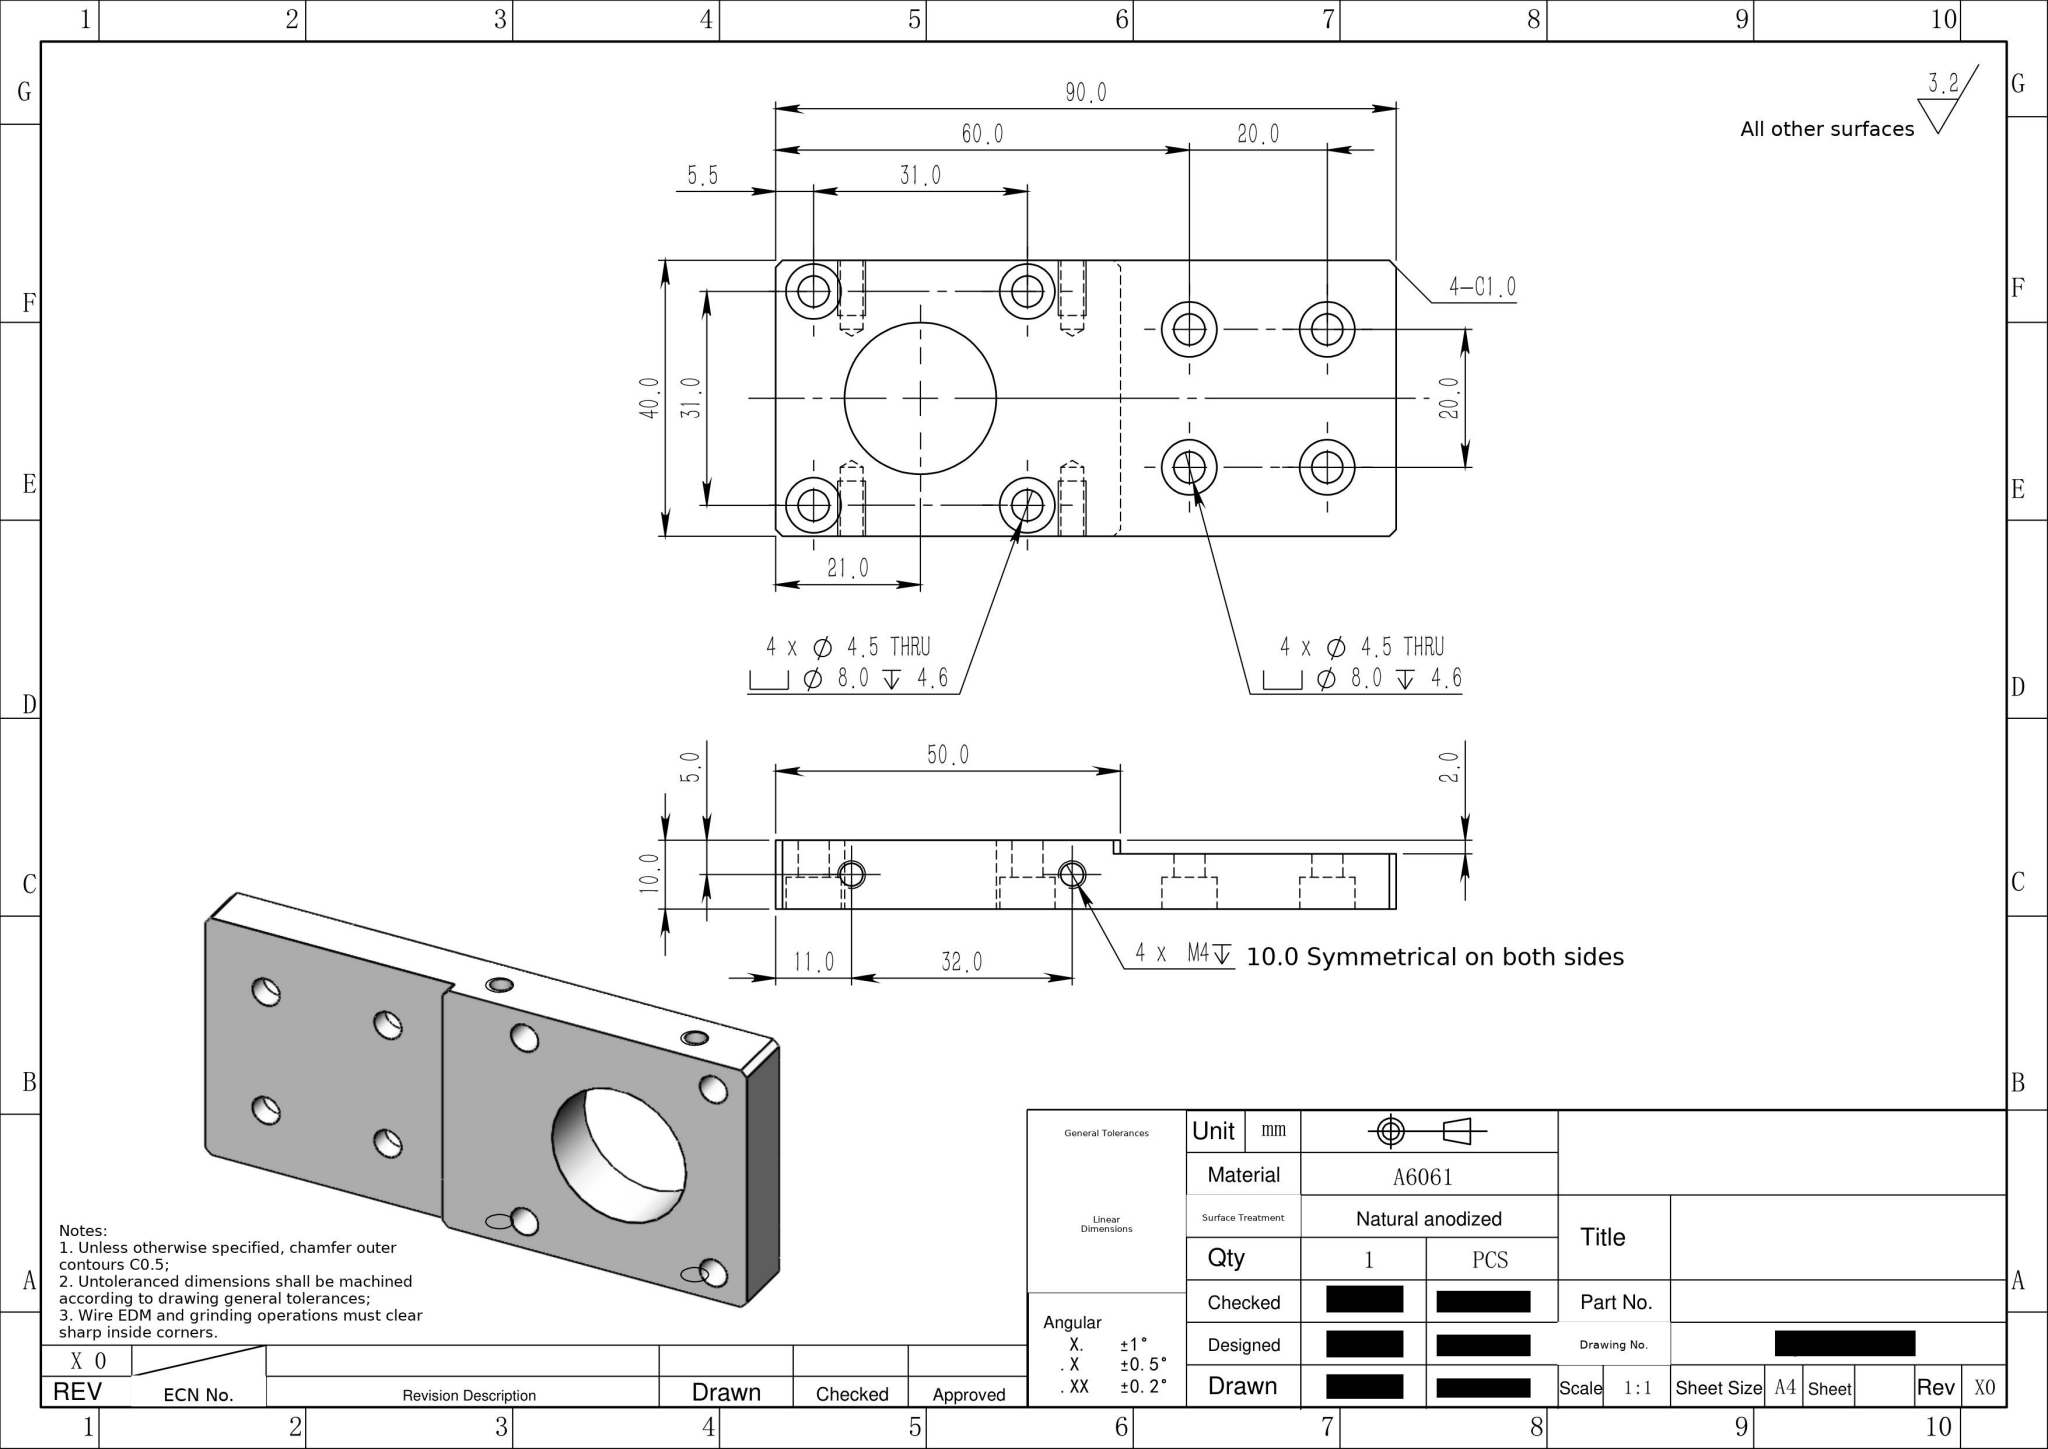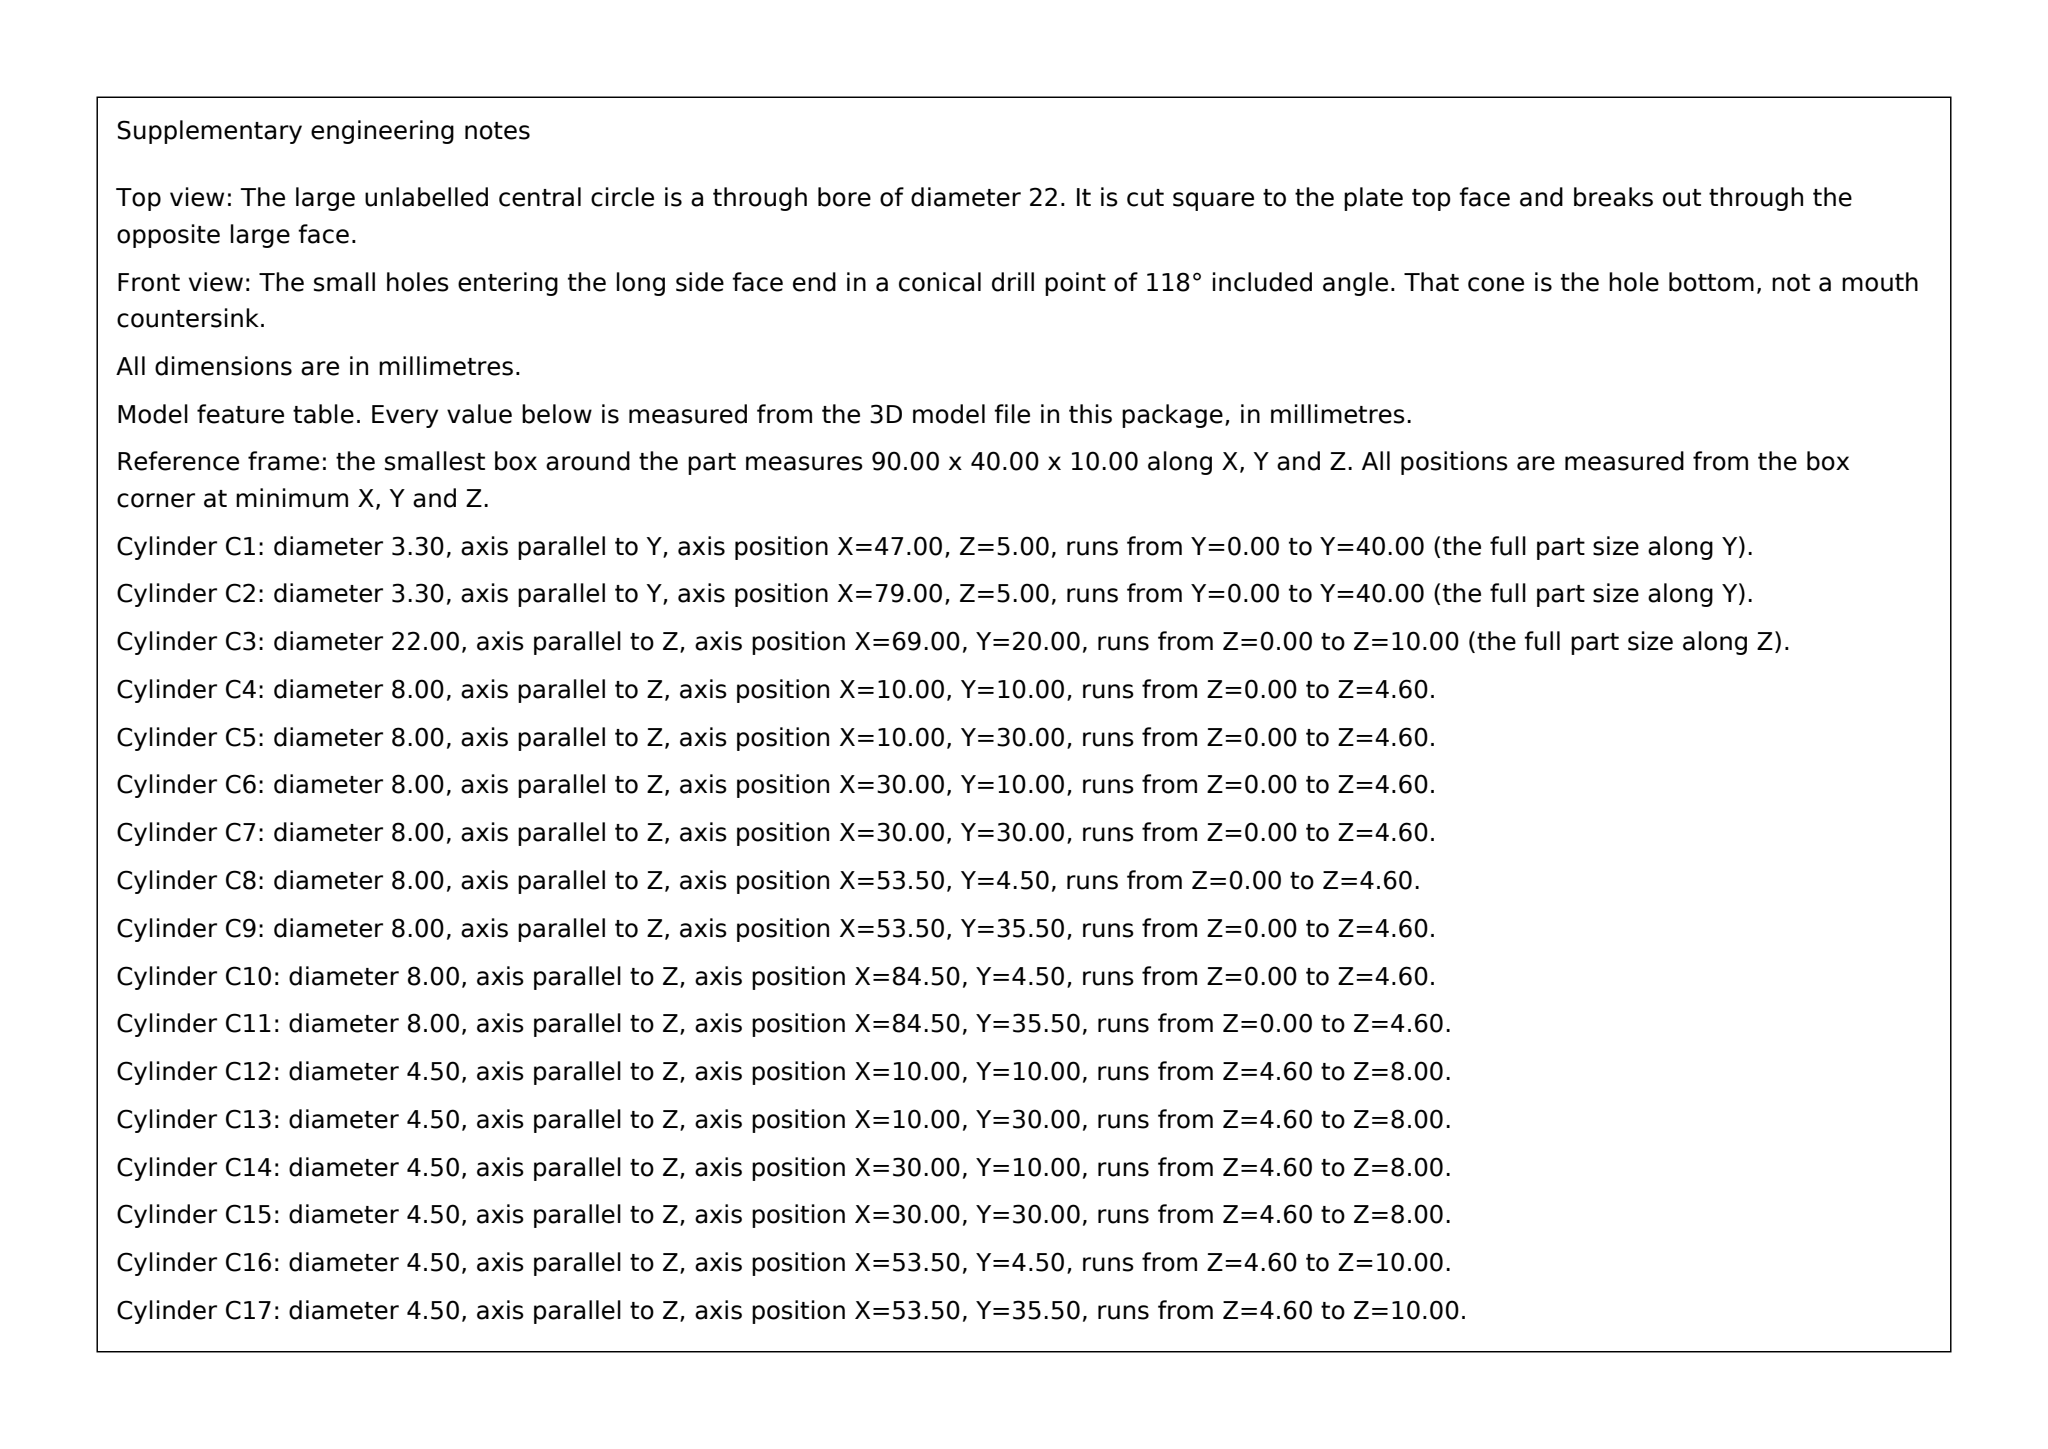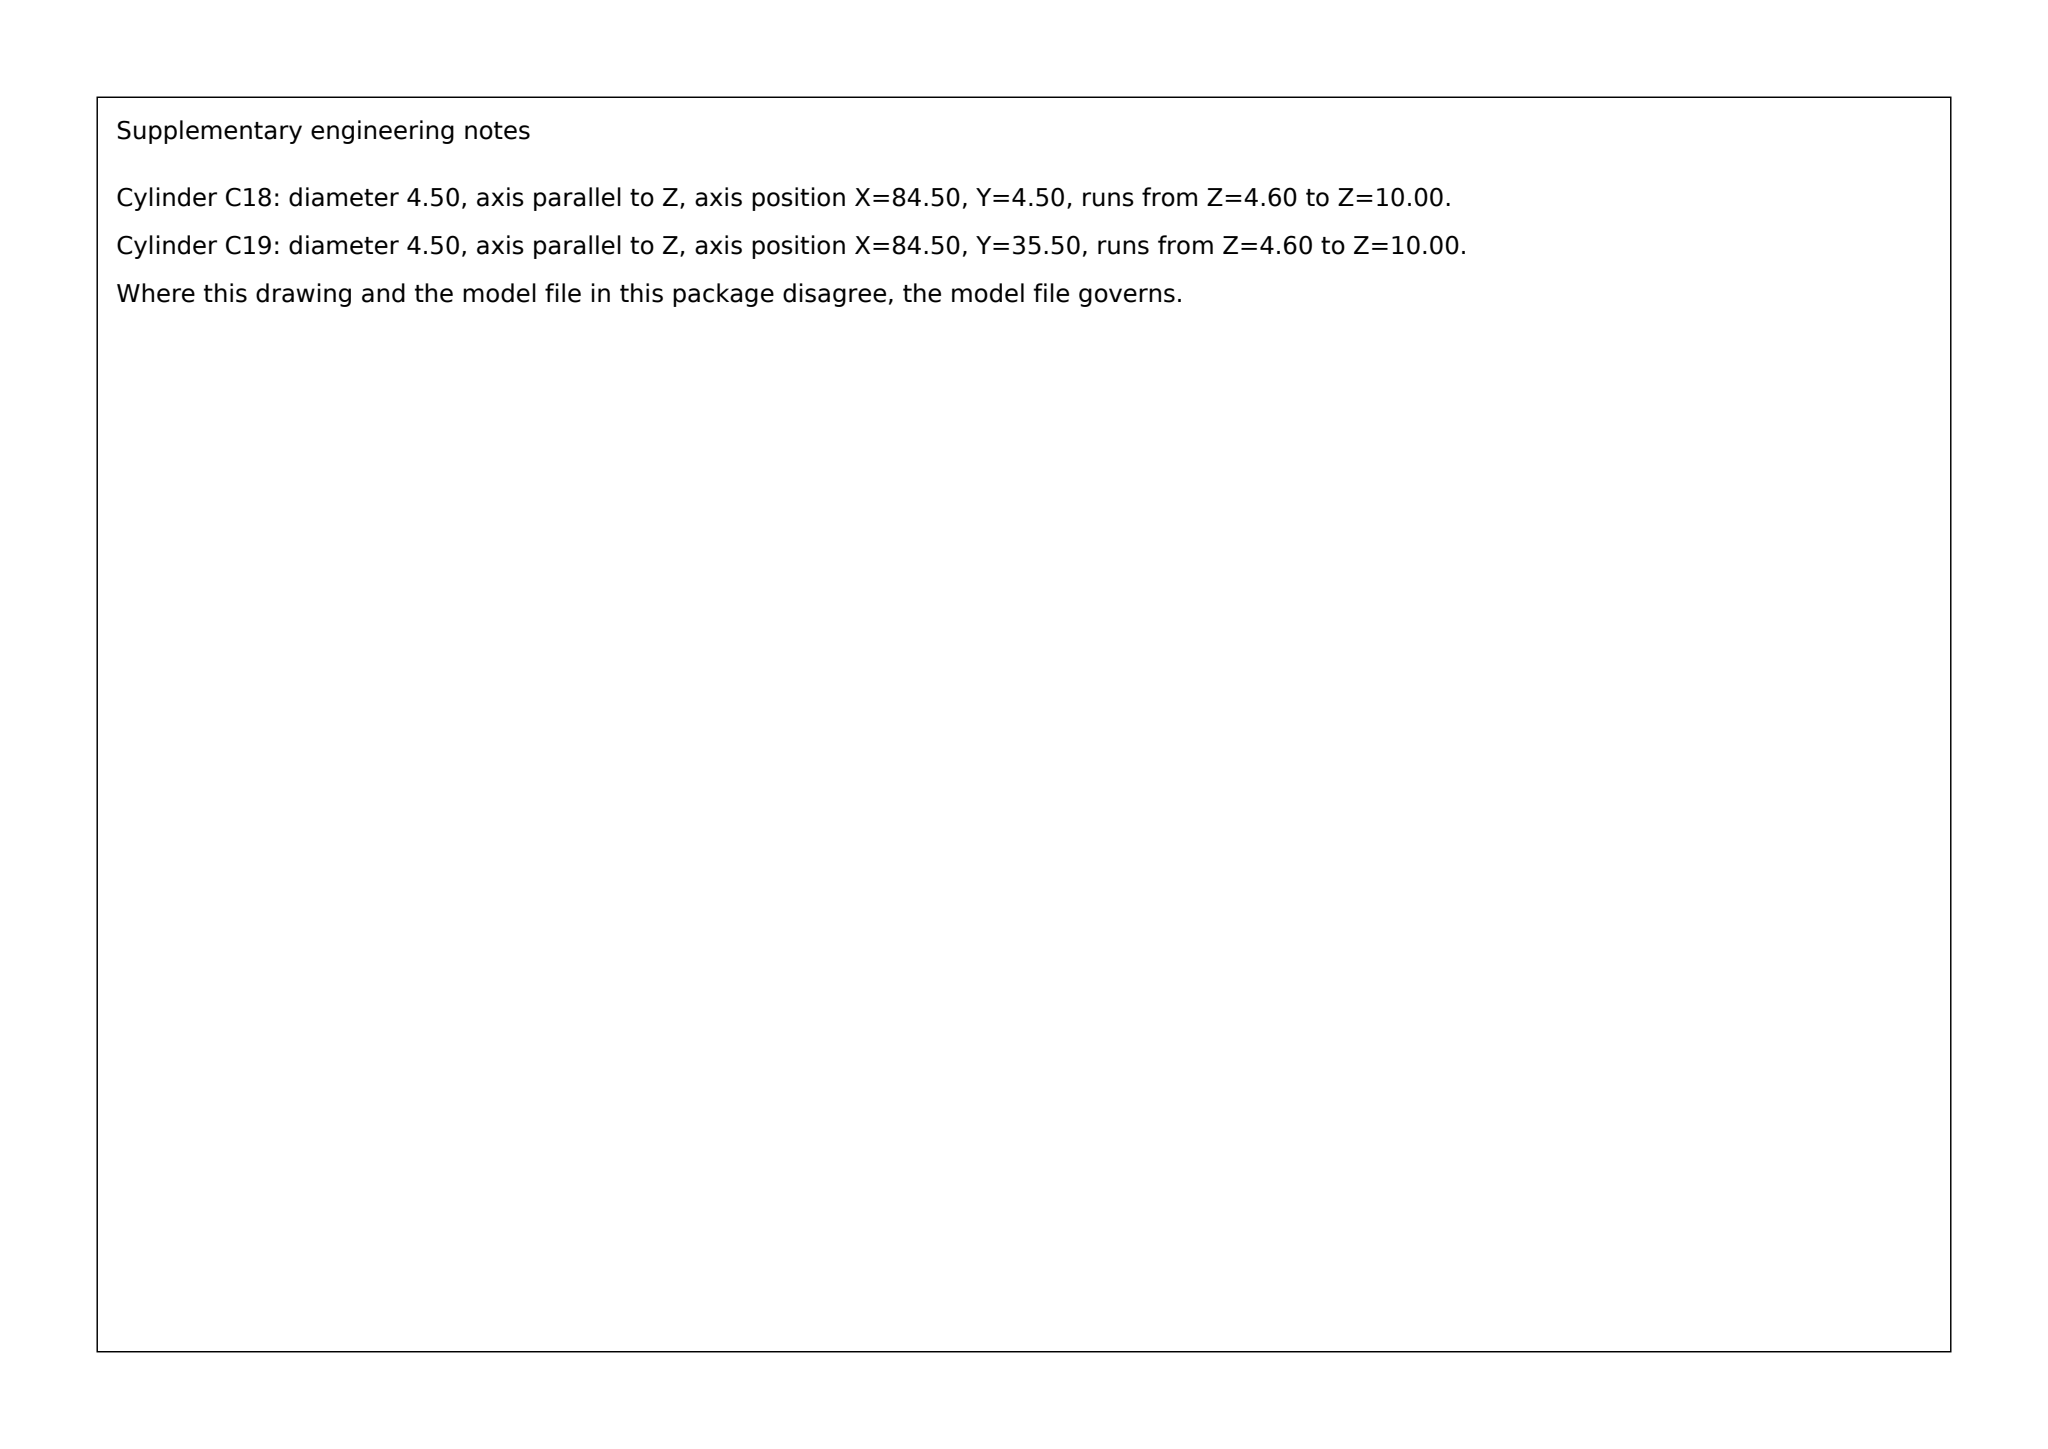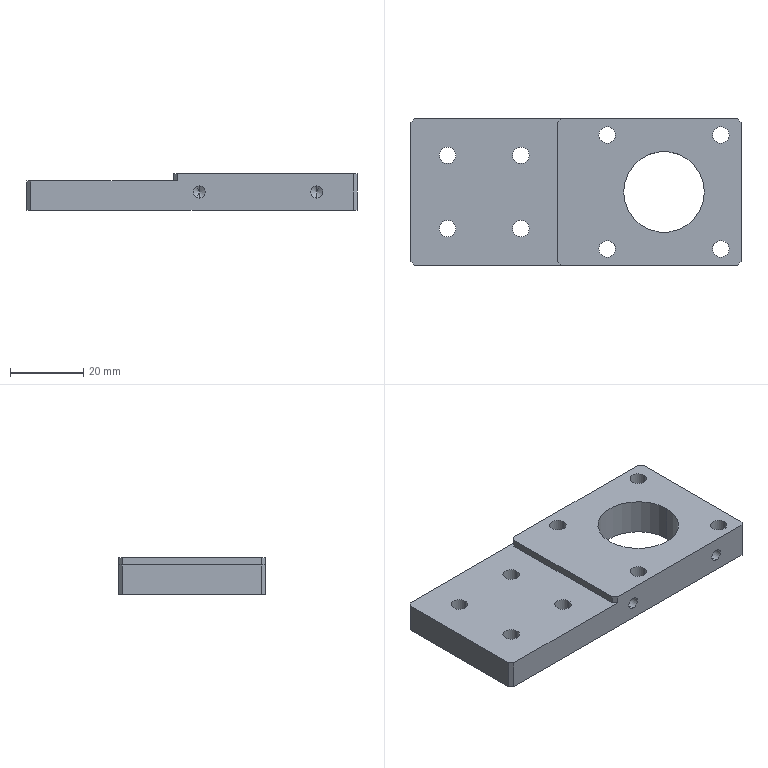Part | SolidWorks | mm | 1 solid | 72 faces | box 90 x 40 x 10 mm | volume 26216 mm3 | cylinder 42 | plane 22 | cone 8 | commonest cylinder face diameters 8 x16 4.5 x16 3.3 x8 22 x2
build123d program:
from build123d import *

# Parameters (mm, degrees)
SKETCH1_W                                            = 90
SKETCH1_H                                            = 40
BOSS_EXTRUDE1_DEPTH                                  = 5
SKETCH2_W                                            = 40
SKETCH2_H                                            = 40
CUT_EXTRUDE1_DEPTH                                   = 2
HOLE_SIZE_ACCORDING_TO_TYPE_3_OF_HEXAGON_D           = 4.5
HOLE_SIZE_ACCORDING_TO_TYPE_3_OF_HEXAGON_CBORE_D     = 8
HOLE_SIZE_ACCORDING_TO_TYPE_3_OF_HEXAGON_CBORE_DEPTH = 4.6
SKETCH7_R                                            = 11
CUT_EXTRUDE2_DEPTH                                   = 51.249
HOLE_SIZE_ACCORDING_TO_TYPE_3_OF_HEX_2_D             = 4.5
HOLE_SIZE_ACCORDING_TO_TYPE_3_OF_HEX_2_CBORE_D       = 8
HOLE_SIZE_ACCORDING_TO_TYPE_3_OF_HEX_2_CBORE_DEPTH   = 4.6
M4_TAPPED_HOLE1_AT_2_COUNT                           = 2
M4_TAPPED_HOLE1_AT_2_PITCH                           = 32
CHAMFER1_SIZE                                        = 1


with BuildPart() as part:
    # Sketch1 → Boss-Extrude1 (new, symmetric)
    with BuildSketch(Plane.XY):
        Rectangle(SKETCH1_W, SKETCH1_H)
    extrude(amount=BOSS_EXTRUDE1_DEPTH, both=True)

    # Sketch2 → Cut-Extrude1 (cut)
    with BuildSketch(Plane.XY.offset(5)):
        with Locations((-25, 0)):
            Rectangle(SKETCH2_W, SKETCH2_H)
    extrude(amount=-CUT_EXTRUDE1_DEPTH, mode=Mode.SUBTRACT)

    # Hole Size_According to_Type 3 of Hexagon (through all)
    with Locations(Plane(origin=(0, 0, -5), x_dir=(-1, 0, 0), z_dir=(0, 0, -1))):
        with Locations((15, 10), (35, 10), (35, -10), (15, -10)):
            CounterBoreHole(HOLE_SIZE_ACCORDING_TO_TYPE_3_OF_HEXAGON_D / 2, HOLE_SIZE_ACCORDING_TO_TYPE_3_OF_HEXAGON_CBORE_D / 2, HOLE_SIZE_ACCORDING_TO_TYPE_3_OF_HEXAGON_CBORE_DEPTH)

    # Sketch7 → Cut-Extrude2 (cut, through all)
    with BuildSketch(Plane(origin=(0, 0, -5), x_dir=(-1, 0, 0), z_dir=(0, 0, -1))):
        with Locations((-24, 0)):
            Circle(SKETCH7_R)
    extrude(amount=-CUT_EXTRUDE2_DEPTH, mode=Mode.SUBTRACT)

    # Hole Size_According to_Type 3 of Hex 2 (through all)
    with Locations(Plane(origin=(0, 0, -5), x_dir=(-1, 0, 0), z_dir=(0, 0, -1))):
        with Locations((-39.5, 15.5), (-8.5, 15.5), (-8.5, -15.5), (-39.5, -15.5)):
            CounterBoreHole(HOLE_SIZE_ACCORDING_TO_TYPE_3_OF_HEX_2_D / 2, HOLE_SIZE_ACCORDING_TO_TYPE_3_OF_HEX_2_CBORE_D / 2, HOLE_SIZE_ACCORDING_TO_TYPE_3_OF_HEX_2_CBORE_DEPTH)

    # Sketch11 → M4 Tapped Hole1 (revolve, cut)
    with BuildSketch(Plane(origin=(2, 20, 0), x_dir=(0, 0, 1), z_dir=(1, 0, 0))):
        Polygon((0, 0), (0, 10.991), (1.65, 10), (1.65, 0), align=None)
    m4_tapped_hole1 = revolve(axis=Axis((2, 26.35, 0), (0, -1, 0)), mode=Mode.SUBTRACT)

    # M4 Tapped Hole1 at 2: M4 Tapped Hole1 ×2
    with Locations(*[(i * M4_TAPPED_HOLE1_AT_2_PITCH, 0, 0) for i in range(1, M4_TAPPED_HOLE1_AT_2_COUNT)]):
        add(m4_tapped_hole1, mode=Mode.SUBTRACT)

    # Mirror1: M4 Tapped Hole1 across plane
    add(m4_tapped_hole1.mirror(Plane.ZX), mode=Mode.SUBTRACT)

    # Mirror1 copy 1 sketch → Mirror1 copy 1 (revolve, cut)
    with BuildSketch(Plane(origin=(34, -20, 0), x_dir=(0, 0, 1), z_dir=(1, 0, 0))):
        Polygon((0, 0), (0, -10.991), (1.65, -10), (1.65, 0), align=None)
    revolve(axis=Axis((34, -26.35, 0), (0, -1, 0)), mode=Mode.SUBTRACT)

    # Chamfer1
    chamfer1_edges = [part.edges().sort_by_distance(p)[0] for p in [
        (-45, 20, -1),
        (-45, -20, -1),
        (-5, 20, 4),
        (-5, -20, 4),
        (45, 20, 0),
        (45, -20, 0),
    ]]
    chamfer(chamfer1_edges, length=CHAMFER1_SIZE)


solid = part.part